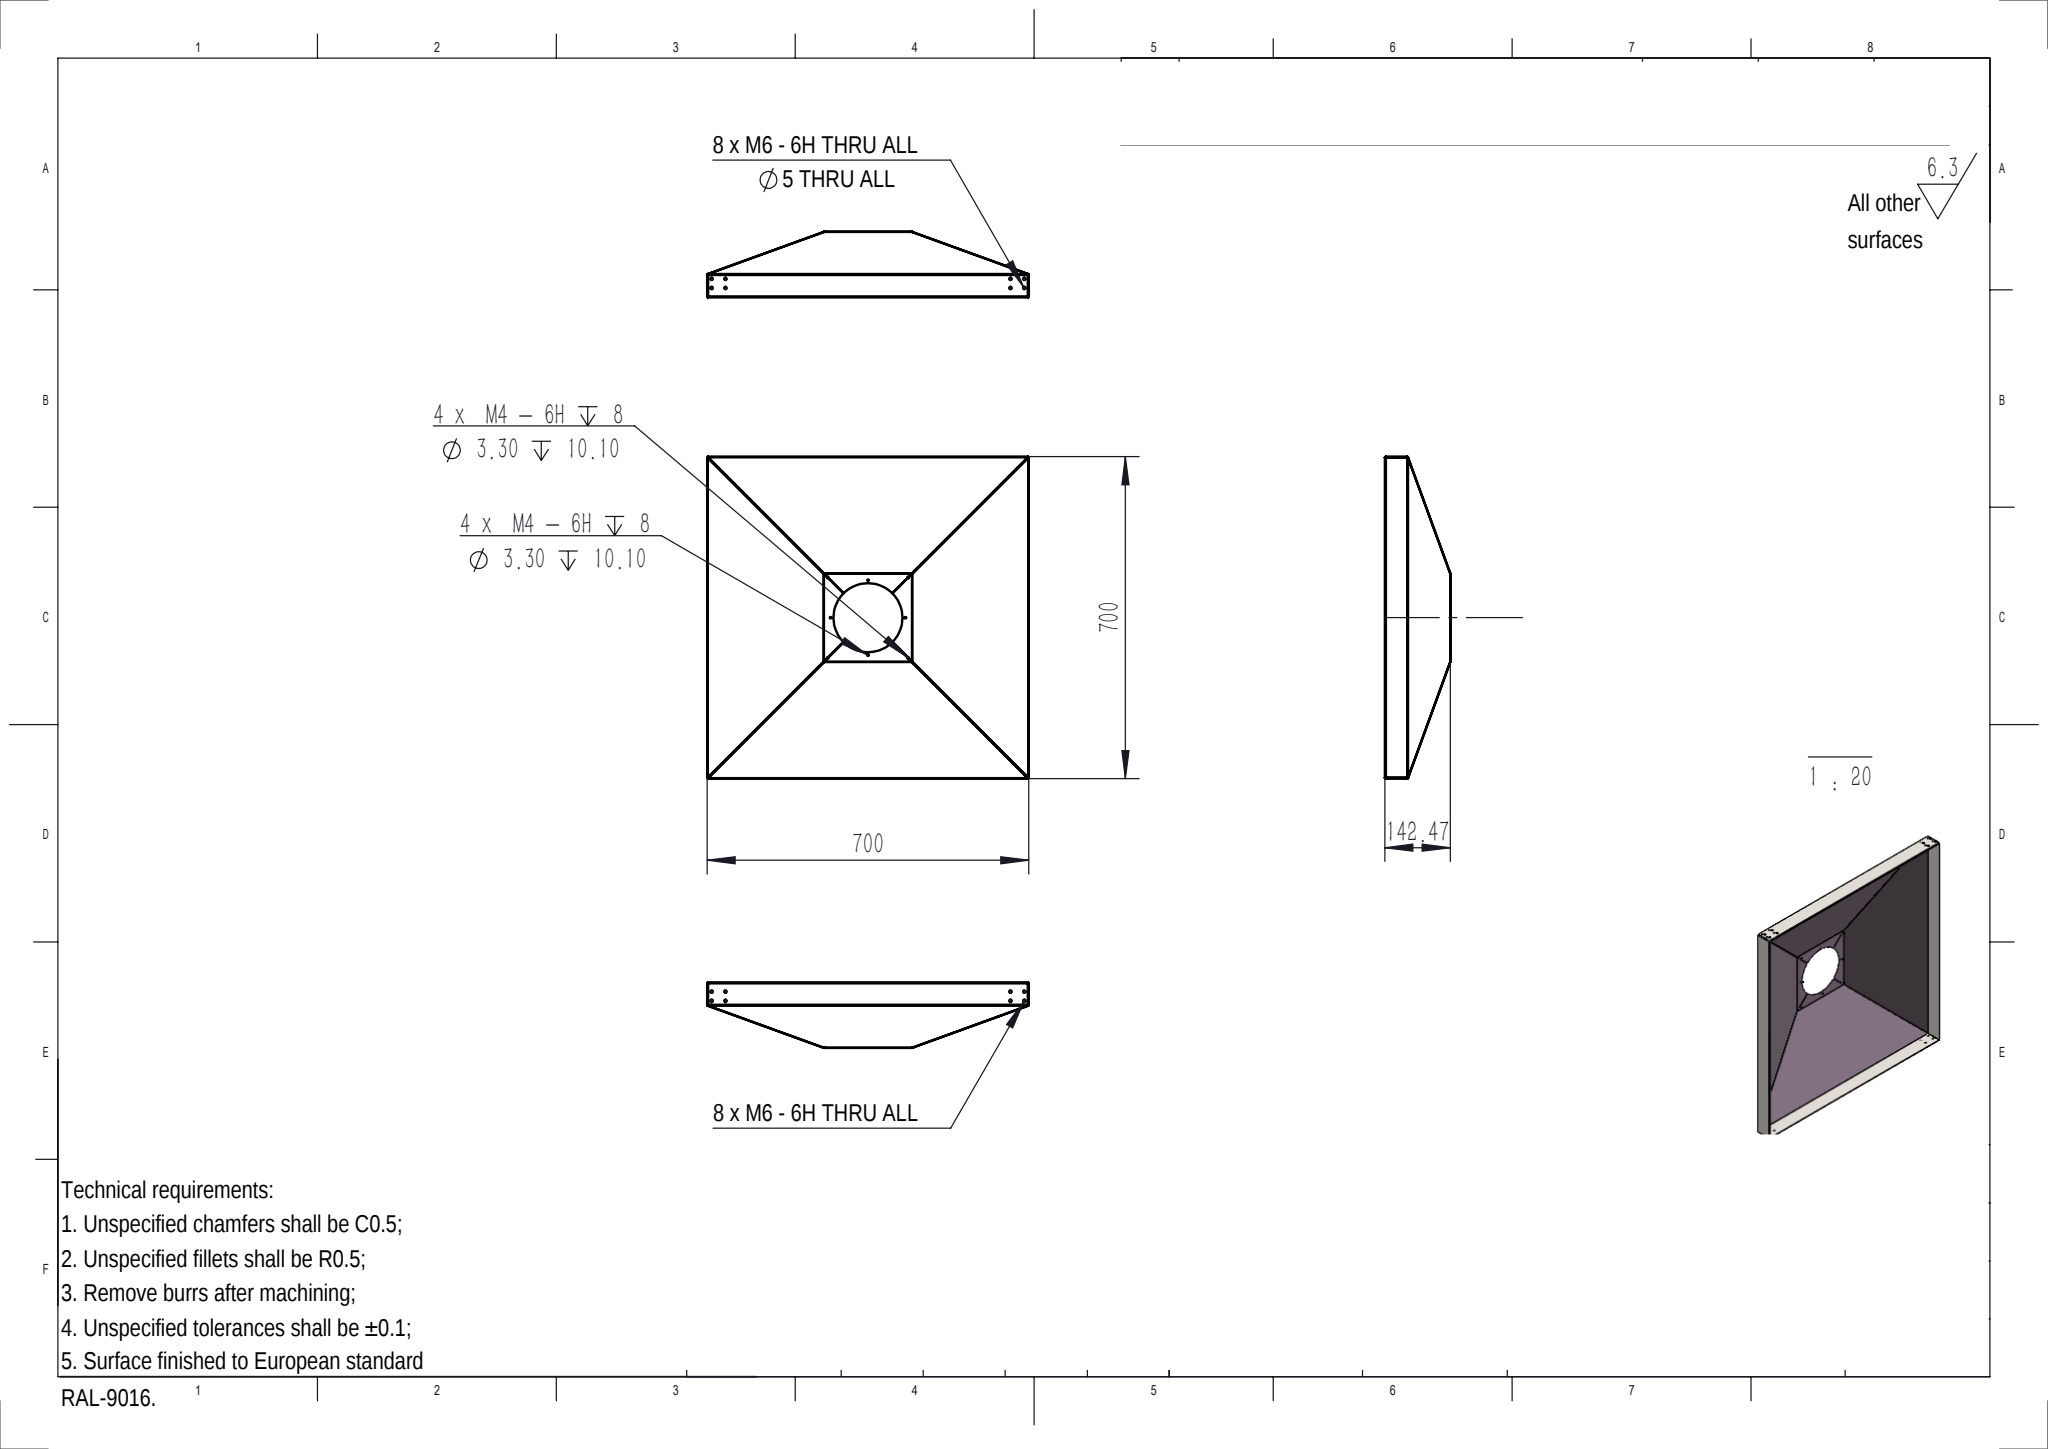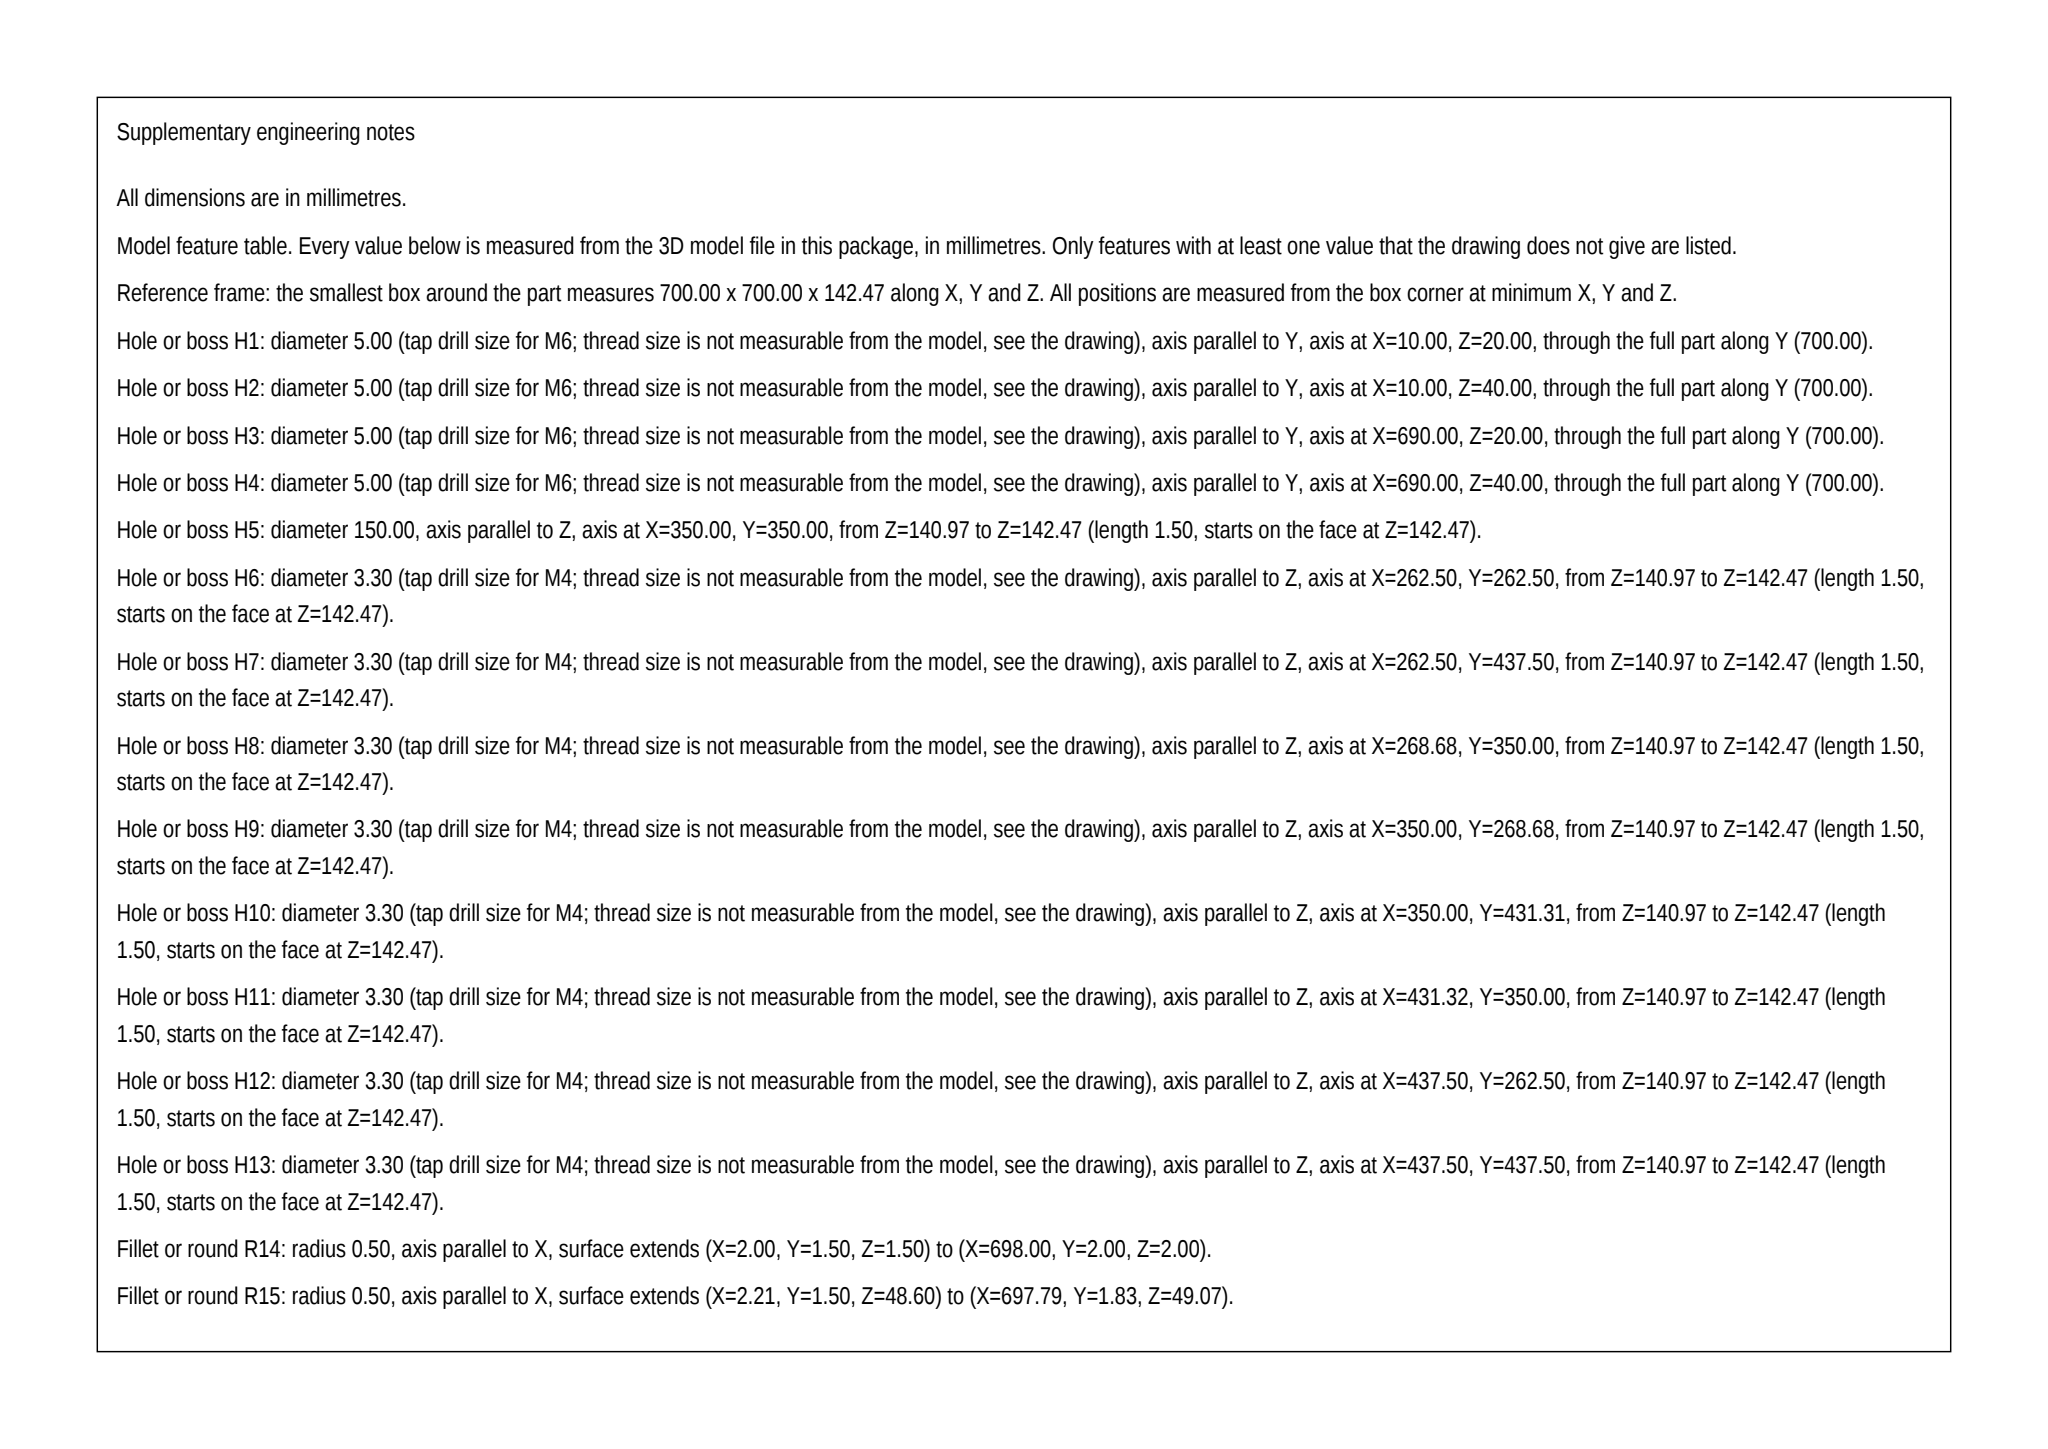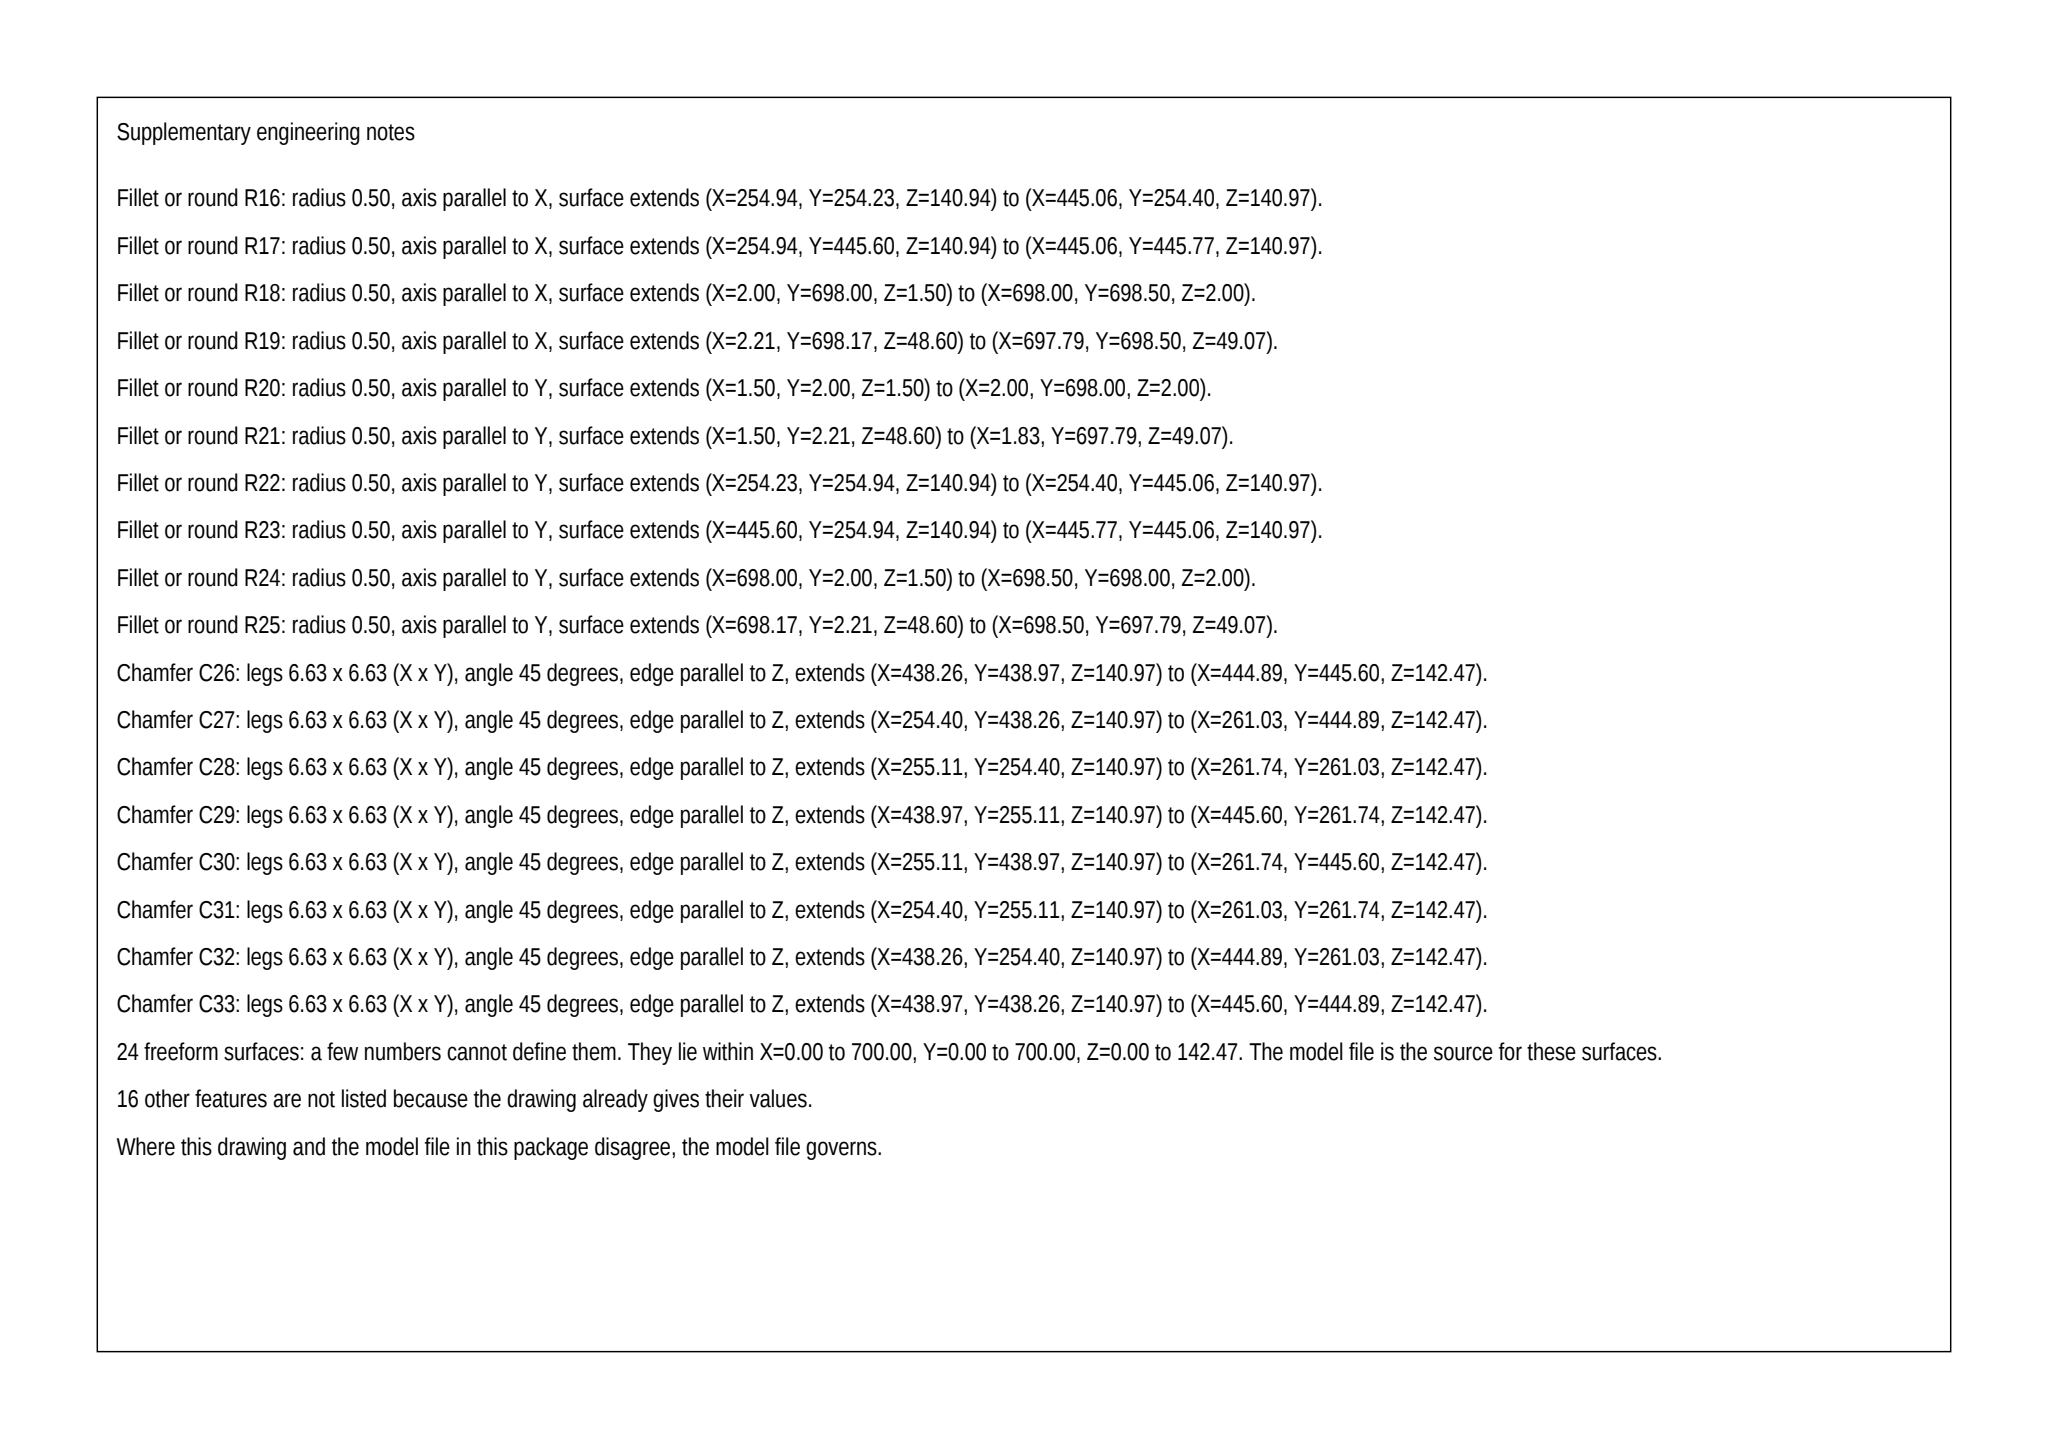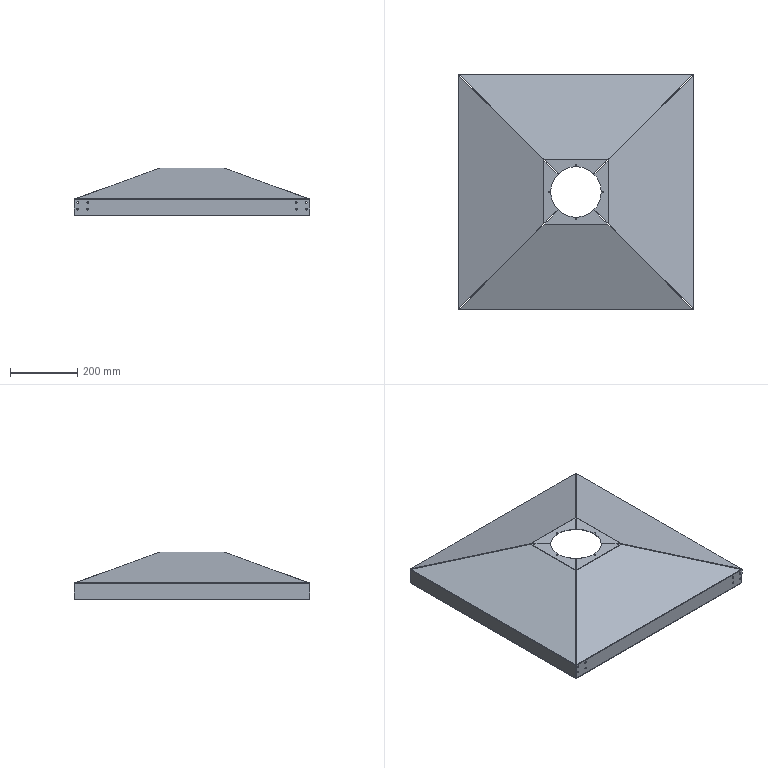Part | SolidWorks | mm | 1 solid | 167 faces | box 700 x 700 x 142.47 mm | volume 952224 mm3 | cylinder 81 | plane 62 | spline 24 | commonest cylinder face diameters 5 x32 3.3 x20 4 x12 1 x12 150 x5